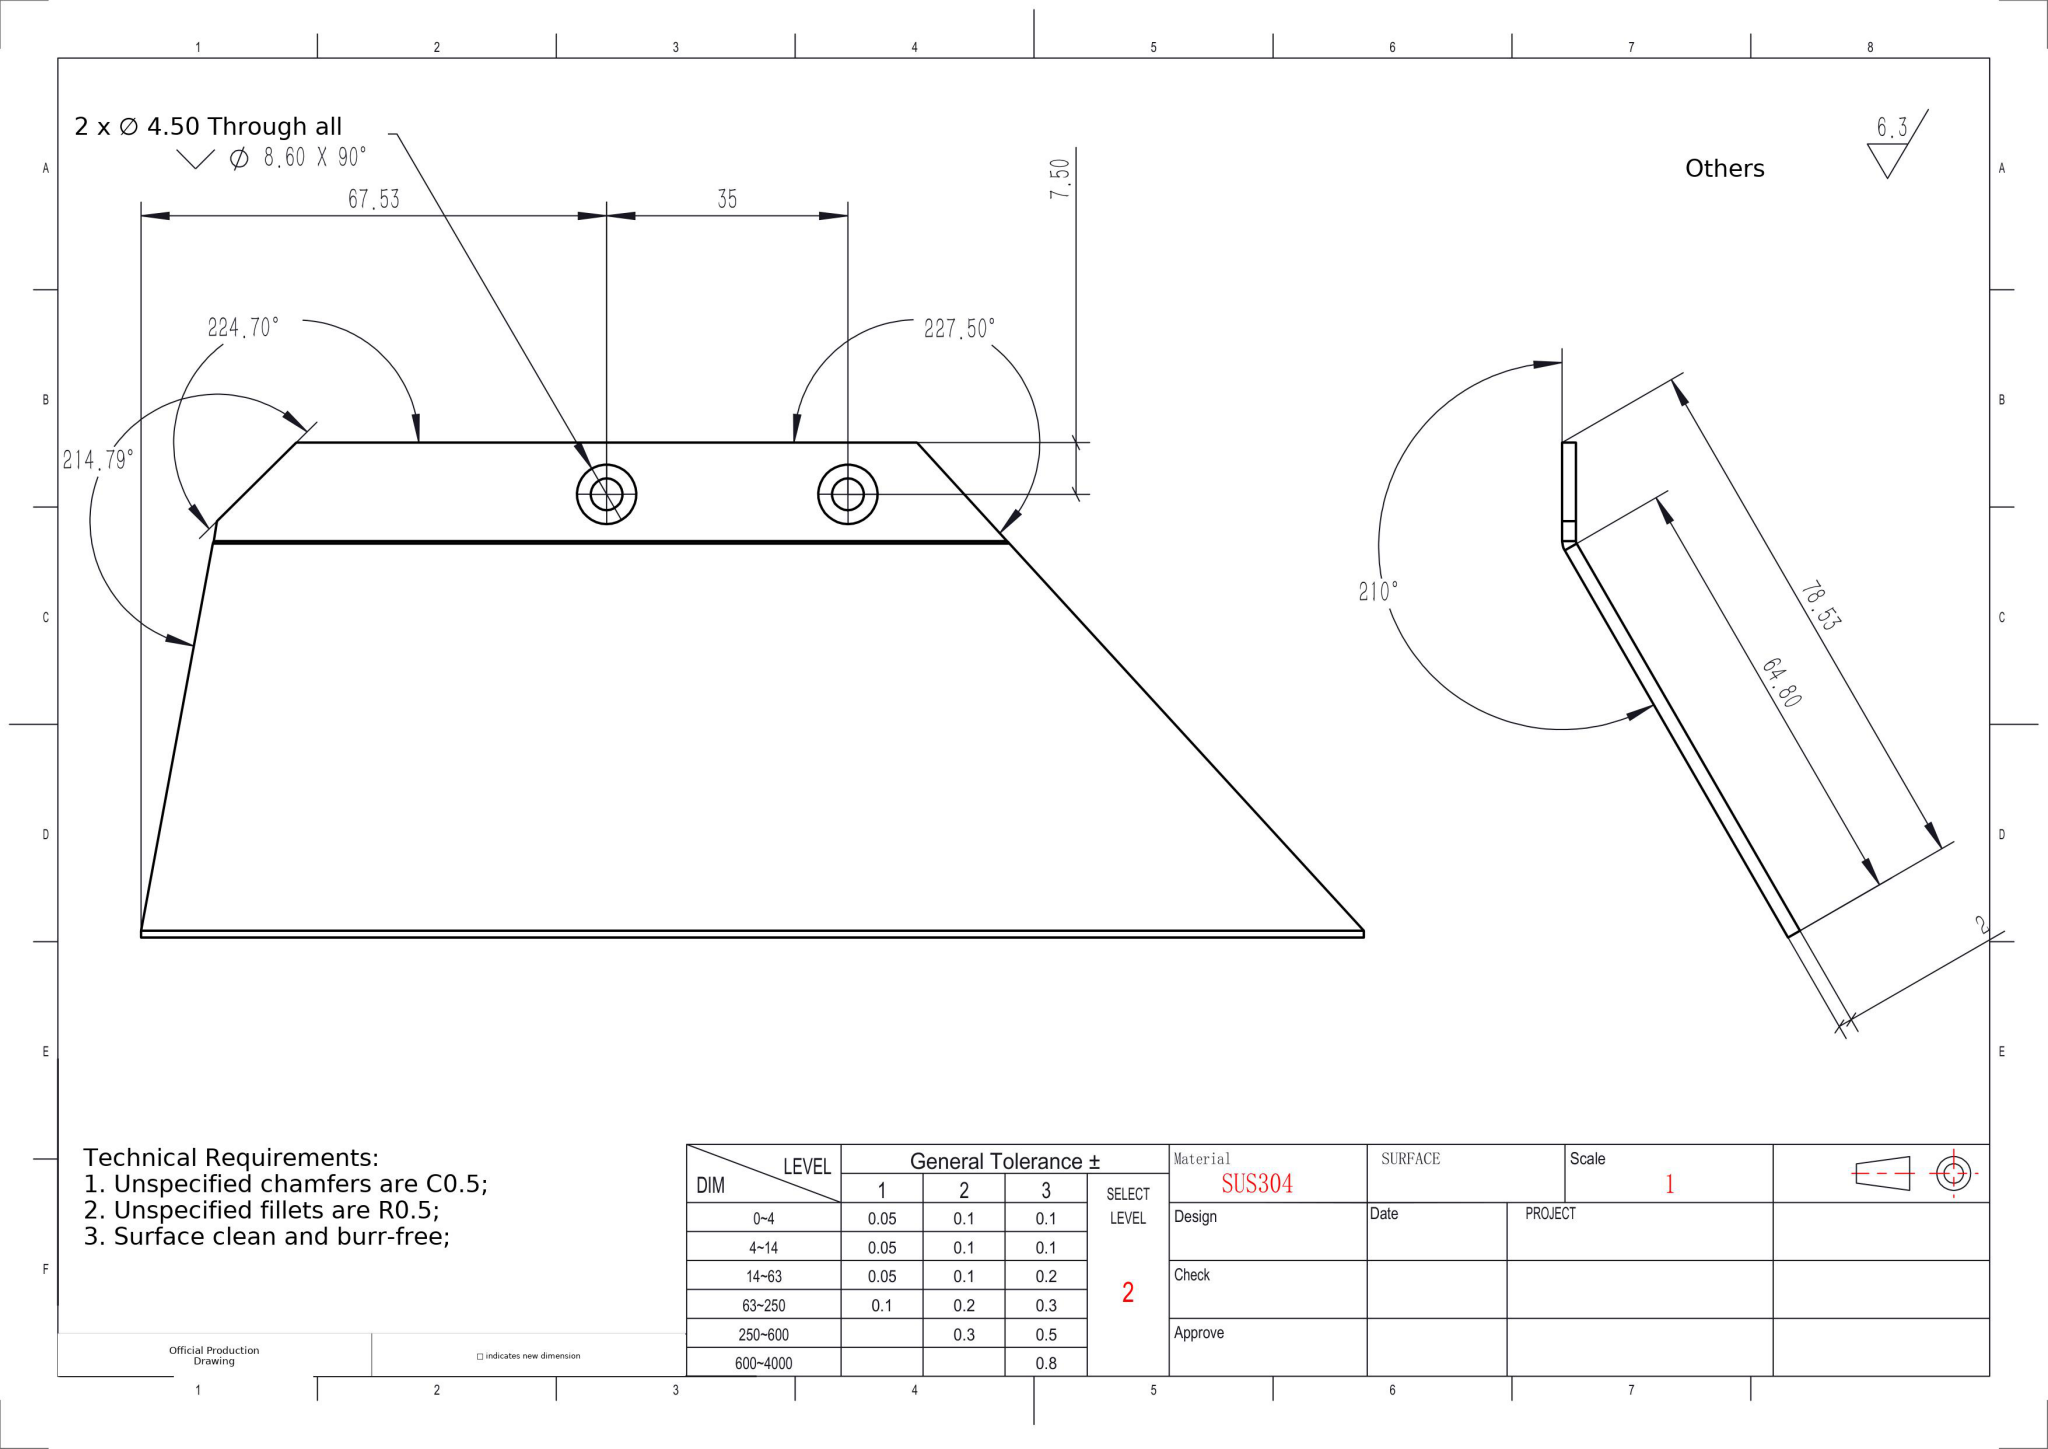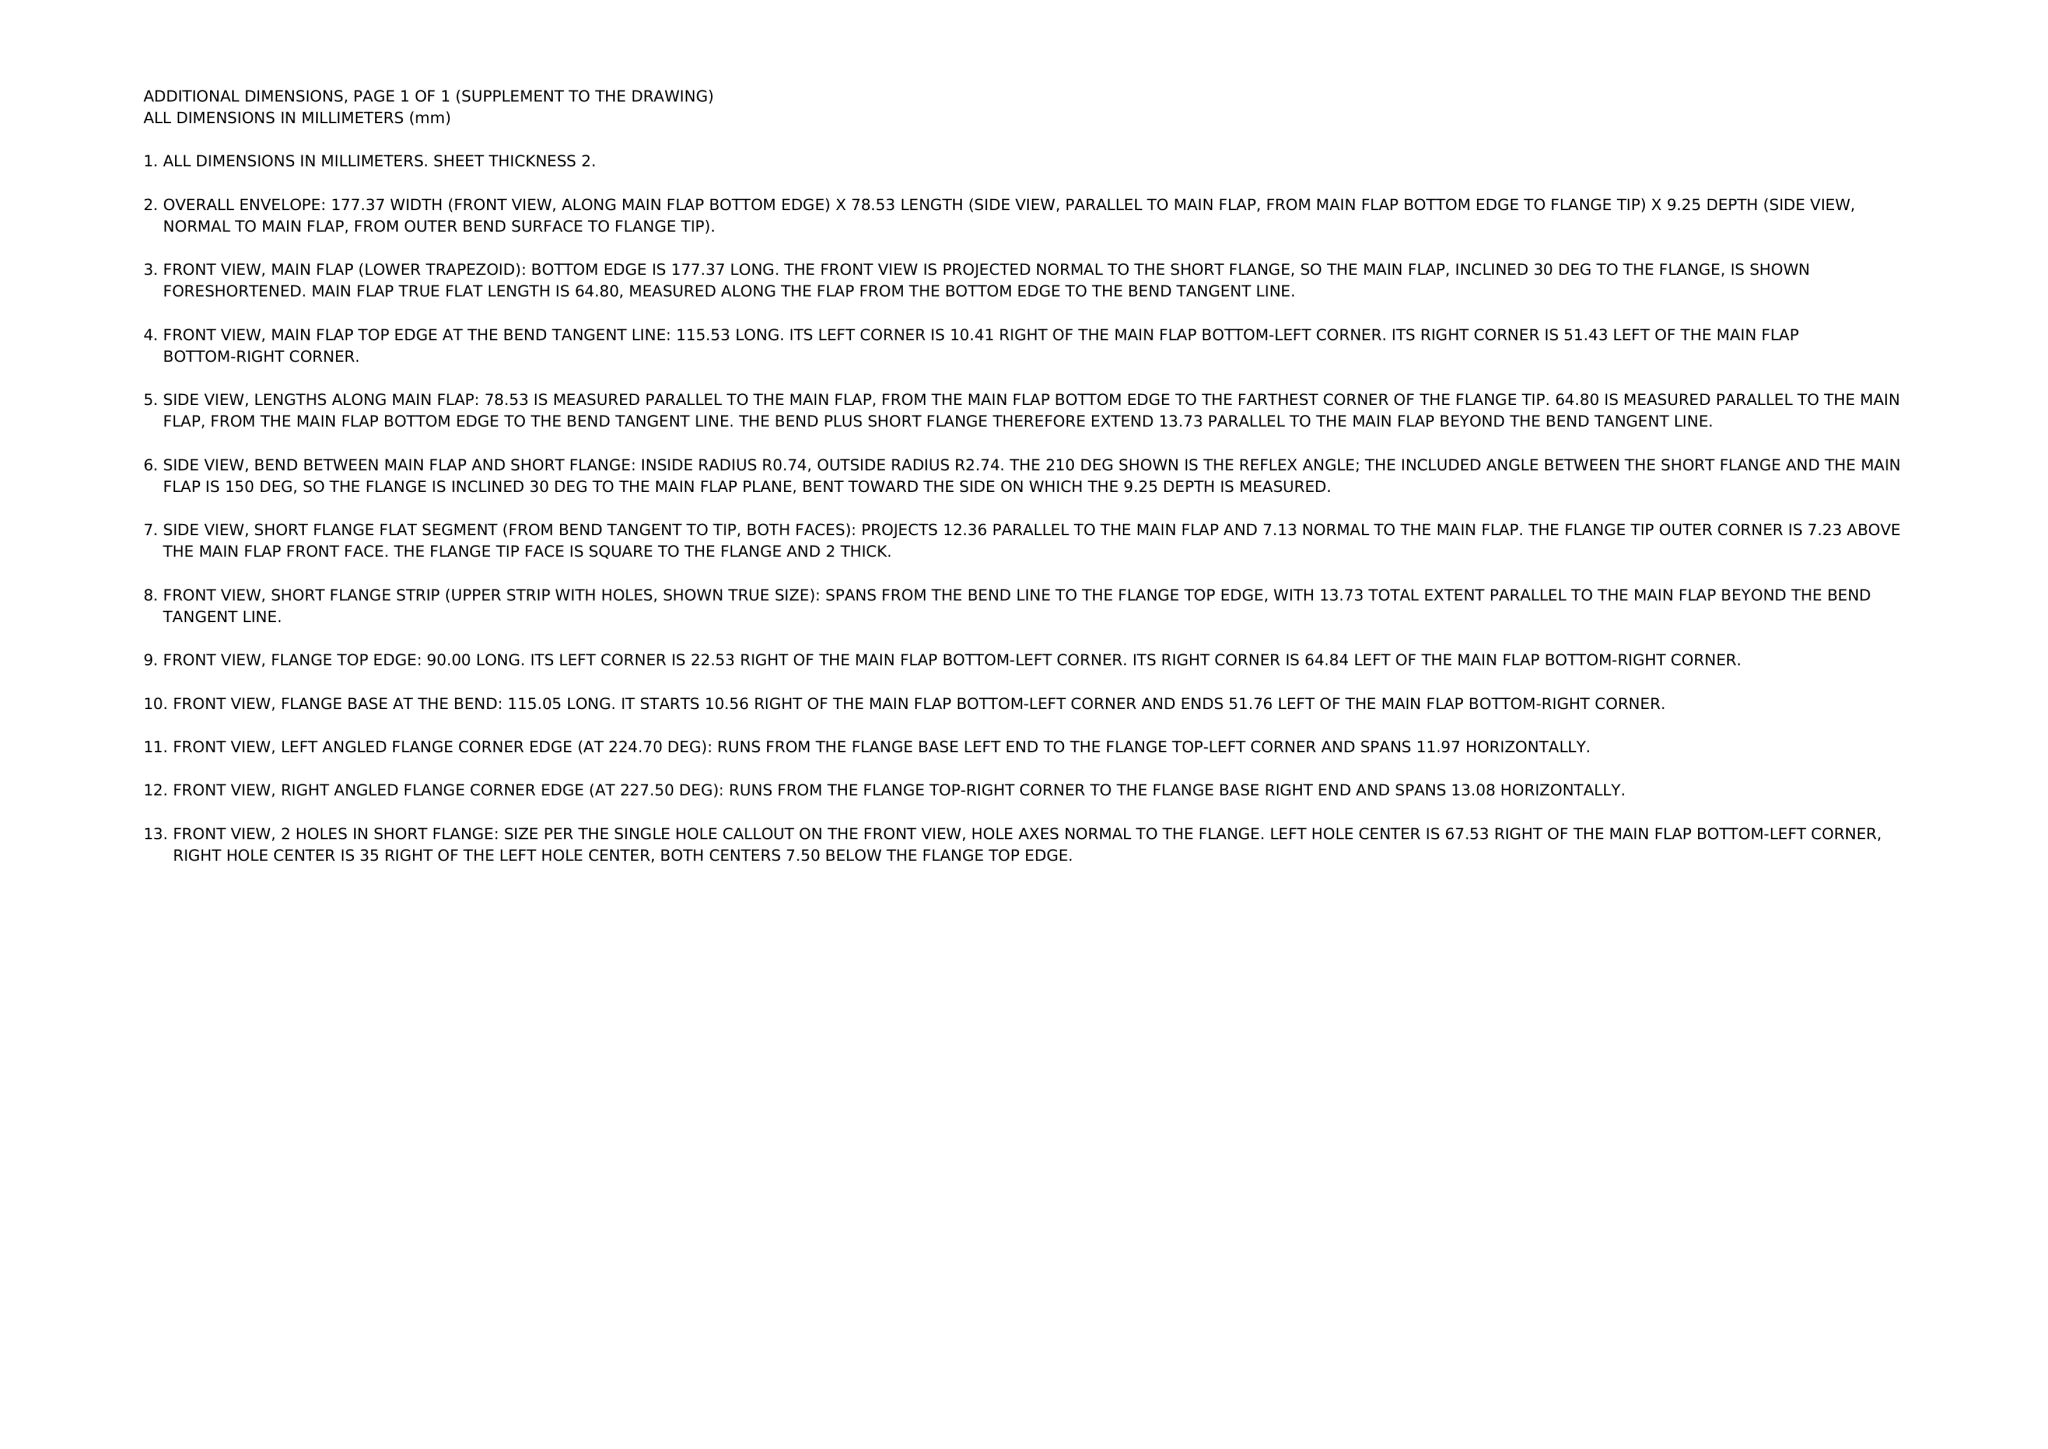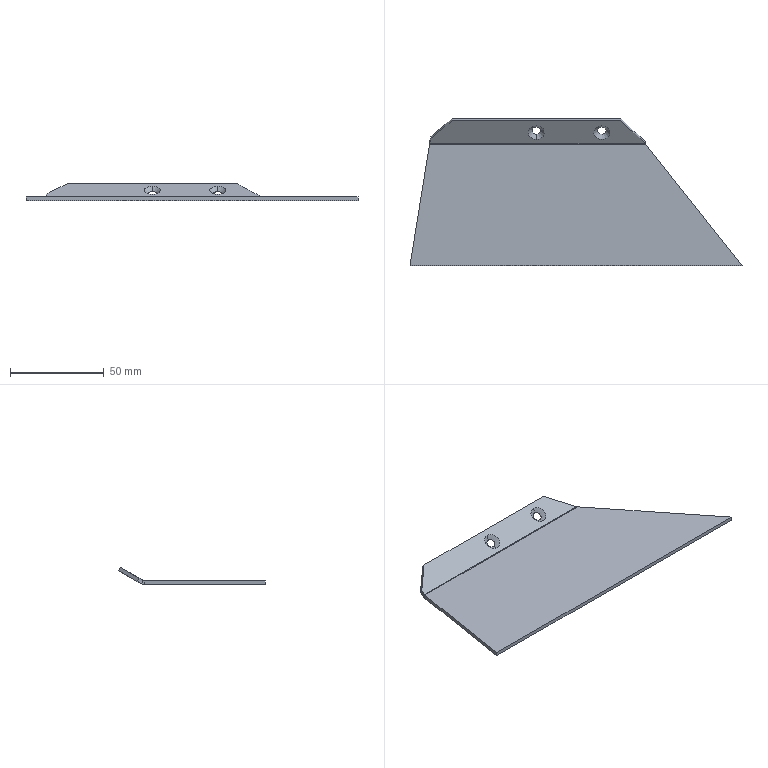Part | NX | mm | 1 solid | 19 faces | box 177.37 x 78.53 x 9.23 mm | volume 22003 mm3 | plane 11 | cone 4 | cylinder 2 | spline 2 | commonest cylinder face diameters 5.473 x1 1.473 x1
STEP:
#1=COLOUR_RGB('',0.698,0.698,0.698);
#2=FILL_AREA_STYLE_COLOUR('',#1);
#3=FILL_AREA_STYLE('',(#2));
#4=SURFACE_STYLE_FILL_AREA(#3);
#5=SURFACE_SIDE_STYLE('',(#4));
#6=SURFACE_STYLE_USAGE(.BOTH.,#5);
#7=PRESENTATION_STYLE_ASSIGNMENT((#6));
#8=CARTESIAN_POINT('',(25.164,41.523,2.9));
#9=VERTEX_POINT('',#8);
#10=CARTESIAN_POINT('',(25.164,37.539,0.6));
#11=VERTEX_POINT('',#10);
#12=CARTESIAN_POINT('',(25.164,39.531,1.75));
#13=DIRECTION('',(0.,-0.5,0.866));
#14=DIRECTION('',(0.,-0.866,-0.5));
#15=AXIS2_PLACEMENT_3D('',#12,#13,#14);
#16=CIRCLE('',#15,2.3);
#17=EDGE_CURVE('',#9,#11,#16,.T.);
#18=ORIENTED_EDGE('',*,*,#17,.F.);
#19=CARTESIAN_POINT('',(25.164,42.255,5.632));
#20=VERTEX_POINT('',#19);
#21=CARTESIAN_POINT('',(25.164,42.255,5.632));
#22=DIRECTION('',(0.,0.2588,0.9659));
#23=VECTOR('',#22,1000.);
#24=LINE('',#21,#23);
#25=EDGE_CURVE('',#9,#20,#24,.T.);
#26=ORIENTED_EDGE('',*,*,#25,.T.);
#27=CARTESIAN_POINT('',(25.164,34.807,1.332));
#28=VERTEX_POINT('',#27);
#29=CARTESIAN_POINT('',(25.164,38.531,3.482));
#30=DIRECTION('',(0.,-0.5,0.866));
#31=DIRECTION('',(0.,-0.866,-0.5));
#32=AXIS2_PLACEMENT_3D('',#29,#30,#31);
#33=CIRCLE('',#32,4.3);
#34=EDGE_CURVE('',#20,#28,#33,.T.);
#35=ORIENTED_EDGE('',*,*,#34,.T.);
#36=CARTESIAN_POINT('',(25.164,34.807,1.332));
#37=DIRECTION('',(0.,-0.9659,0.2588));
#38=VECTOR('',#37,1000.);
#39=LINE('',#36,#38);
#40=EDGE_CURVE('',#11,#28,#39,.T.);
#41=ORIENTED_EDGE('',*,*,#40,.F.);
#42=EDGE_LOOP('',(#18,#26,#35,#41));
#43=FACE_OUTER_BOUND('',#42,.T.);
#44=CARTESIAN_POINT('',(25.164,38.531,3.482));
#45=DIRECTION('',(0.,-0.5,0.866));
#46=DIRECTION('',(0.,-0.866,-0.5));
#47=AXIS2_PLACEMENT_3D('',#44,#45,#46);
#48=CONICAL_SURFACE('',#47,4.3,0.7854);
#49=ADVANCED_FACE('',(#43),#48,.F.);
#50=CARTESIAN_POINT('',(-9.836,41.523,2.9));
#51=VERTEX_POINT('',#50);
#52=CARTESIAN_POINT('',(-9.836,37.539,0.6));
#53=VERTEX_POINT('',#52);
#54=CARTESIAN_POINT('',(-9.836,39.531,1.75));
#55=DIRECTION('',(0.,-0.5,0.866));
#56=DIRECTION('',(0.,-0.866,-0.5));
#57=AXIS2_PLACEMENT_3D('',#54,#55,#56);
#58=CIRCLE('',#57,2.3);
#59=EDGE_CURVE('',#51,#53,#58,.T.);
#60=ORIENTED_EDGE('',*,*,#59,.F.);
#61=CARTESIAN_POINT('',(-9.836,42.255,5.632));
#62=VERTEX_POINT('',#61);
#63=CARTESIAN_POINT('',(-9.836,42.255,5.632));
#64=DIRECTION('',(0.,0.2588,0.9659));
#65=VECTOR('',#64,1000.);
#66=LINE('',#63,#65);
#67=EDGE_CURVE('',#51,#62,#66,.T.);
#68=ORIENTED_EDGE('',*,*,#67,.T.);
#69=CARTESIAN_POINT('',(-9.836,34.807,1.332));
#70=VERTEX_POINT('',#69);
#71=CARTESIAN_POINT('',(-9.836,38.531,3.482));
#72=DIRECTION('',(0.,-0.5,0.866));
#73=DIRECTION('',(0.,-0.866,-0.5));
#74=AXIS2_PLACEMENT_3D('',#71,#72,#73);
#75=CIRCLE('',#74,4.3);
#76=EDGE_CURVE('',#62,#70,#75,.T.);
#77=ORIENTED_EDGE('',*,*,#76,.T.);
#78=CARTESIAN_POINT('',(-9.836,34.807,1.332));
#79=DIRECTION('',(0.,-0.9659,0.2588));
#80=VECTOR('',#79,1000.);
#81=LINE('',#78,#80);
#82=EDGE_CURVE('',#53,#70,#81,.T.);
#83=ORIENTED_EDGE('',*,*,#82,.F.);
#84=EDGE_LOOP('',(#60,#68,#77,#83));
#85=FACE_OUTER_BOUND('',#84,.T.);
#86=CARTESIAN_POINT('',(-9.836,38.531,3.482));
#87=DIRECTION('',(0.,-0.5,0.866));
#88=DIRECTION('',(0.,-0.866,-0.5));
#89=AXIS2_PLACEMENT_3D('',#86,#87,#88);
#90=CONICAL_SURFACE('',#89,4.3,0.7854);
#91=ADVANCED_FACE('',(#85),#90,.F.);
#92=CARTESIAN_POINT('',(-77.367,-32.5,-2.));
#93=VERTEX_POINT('',#92);
#94=CARTESIAN_POINT('',(-66.958,32.303,-2.));
#95=VERTEX_POINT('',#94);
#96=CARTESIAN_POINT('',(-70.332,11.298,-2.));
#97=DIRECTION('',(0.1586,0.9873,0.));
#98=VECTOR('',#97,1000.);
#99=LINE('',#96,#98);
#100=EDGE_CURVE('',#93,#95,#99,.T.);
#101=ORIENTED_EDGE('',*,*,#100,.T.);
#102=CARTESIAN_POINT('',(48.575,32.303,-2.));
#103=VERTEX_POINT('',#102);
#104=CARTESIAN_POINT('',(-100.,32.303,-2.));
#105=DIRECTION('',(1.,0.,0.));
#106=VECTOR('',#105,1000.);
#107=LINE('',#104,#106);
#108=EDGE_CURVE('',#95,#103,#107,.T.);
#109=ORIENTED_EDGE('',*,*,#108,.T.);
#110=CARTESIAN_POINT('',(100.,-32.5,-2.));
#111=VERTEX_POINT('',#110);
#112=CARTESIAN_POINT('',(45.534,36.134,-2.));
#113=DIRECTION('',(-0.6216,0.7833,0.));
#114=VECTOR('',#113,1000.);
#115=LINE('',#112,#114);
#116=EDGE_CURVE('',#111,#103,#115,.T.);
#117=ORIENTED_EDGE('',*,*,#116,.F.);
#118=CARTESIAN_POINT('',(-100.,-32.5,-2.));
#119=DIRECTION('',(1.,0.,0.));
#120=VECTOR('',#119,1000.);
#121=LINE('',#118,#120);
#122=EDGE_CURVE('',#93,#111,#121,.T.);
#123=ORIENTED_EDGE('',*,*,#122,.F.);
#124=EDGE_LOOP('',(#101,#109,#117,#123));
#125=FACE_OUTER_BOUND('',#124,.T.);
#126=CARTESIAN_POINT('',(0.,0.,-2.));
#127=DIRECTION('',(0.,0.,1.));
#128=DIRECTION('',(1.,0.,0.));
#129=AXIS2_PLACEMENT_3D('',#126,#127,#128);
#130=PLANE('',#129);
#131=ADVANCED_FACE('',(#125),#130,.F.);
#132=CARTESIAN_POINT('',(-66.958,32.303,-0.));
#133=VERTEX_POINT('',#132);
#134=CARTESIAN_POINT('',(48.575,32.303,0.));
#135=VERTEX_POINT('',#134);
#136=CARTESIAN_POINT('',(-100.,32.303,-0.));
#137=DIRECTION('',(1.,0.,0.));
#138=VECTOR('',#137,1000.);
#139=LINE('',#136,#138);
#140=EDGE_CURVE('',#133,#135,#139,.T.);
#141=ORIENTED_EDGE('',*,*,#140,.F.);
#142=CARTESIAN_POINT('',(-77.367,-32.5,0.));
#143=VERTEX_POINT('',#142);
#144=CARTESIAN_POINT('',(-70.332,11.298,0.));
#145=DIRECTION('',(0.1586,0.9873,0.));
#146=VECTOR('',#145,1000.);
#147=LINE('',#144,#146);
#148=EDGE_CURVE('',#143,#133,#147,.T.);
#149=ORIENTED_EDGE('',*,*,#148,.F.);
#150=CARTESIAN_POINT('',(100.,-32.5,0.));
#151=VERTEX_POINT('',#150);
#152=CARTESIAN_POINT('',(-100.,-32.5,0.));
#153=DIRECTION('',(1.,0.,0.));
#154=VECTOR('',#153,1000.);
#155=LINE('',#152,#154);
#156=EDGE_CURVE('',#143,#151,#155,.T.);
#157=ORIENTED_EDGE('',*,*,#156,.T.);
#158=CARTESIAN_POINT('',(45.534,36.134,0.));
#159=DIRECTION('',(-0.6216,0.7833,0.));
#160=VECTOR('',#159,1000.);
#161=LINE('',#158,#160);
#162=EDGE_CURVE('',#151,#135,#161,.T.);
#163=ORIENTED_EDGE('',*,*,#162,.T.);
#164=EDGE_LOOP('',(#141,#149,#157,#163));
#165=FACE_OUTER_BOUND('',#164,.T.);
#166=CARTESIAN_POINT('',(0.,0.,0.));
#167=DIRECTION('',(0.,0.,1.));
#168=DIRECTION('',(1.,0.,0.));
#169=AXIS2_PLACEMENT_3D('',#166,#167,#168);
#170=PLANE('',#169);
#171=ADVANCED_FACE('',(#165),#170,.T.);
#172=ORIENTED_EDGE('',*,*,#108,.F.);
#173=CARTESIAN_POINT('',(-66.813,33.671,-1.633));
#174=VERTEX_POINT('',#173);
#175=CARTESIAN_POINT('',(-66.958,32.303,-2.));
#176=CARTESIAN_POINT('',(-66.934,32.542,-2.));
#177=CARTESIAN_POINT('',(-66.91,32.781,-1.969));
#178=CARTESIAN_POINT('',(-66.861,33.243,-1.844));
#179=CARTESIAN_POINT('',(-66.837,33.463,-1.753));
#180=CARTESIAN_POINT('',(-66.813,33.671,-1.633));
#181=B_SPLINE_CURVE_WITH_KNOTS('',3,(#175,#176,#177,#178,#179,#180),.UNSPECIFIED.,.F.,.F.,(4,2,4),(0.,0.0007209,0.001442),.UNSPECIFIED.);
#182=EDGE_CURVE('',#95,#174,#181,.T.);
#183=ORIENTED_EDGE('',*,*,#182,.T.);
#184=CARTESIAN_POINT('',(48.237,33.671,-1.633));
#185=VERTEX_POINT('',#184);
#186=CARTESIAN_POINT('',(0.,33.671,-1.633));
#187=DIRECTION('',(1.,0.,0.));
#188=VECTOR('',#187,1000.);
#189=LINE('',#186,#188);
#190=EDGE_CURVE('',#174,#185,#189,.T.);
#191=ORIENTED_EDGE('',*,*,#190,.T.);
#192=CARTESIAN_POINT('',(48.237,33.671,-1.633));
#193=CARTESIAN_POINT('',(48.294,33.463,-1.753));
#194=CARTESIAN_POINT('',(48.35,33.241,-1.845));
#195=CARTESIAN_POINT('',(48.463,32.778,-1.969));
#196=CARTESIAN_POINT('',(48.518,32.542,-2.));
#197=CARTESIAN_POINT('',(48.575,32.303,-2.));
#198=B_SPLINE_CURVE_WITH_KNOTS('',3,(#192,#193,#194,#195,#196,#197),.UNSPECIFIED.,.F.,.F.,(4,2,4),(0.,0.0007368,0.001474),.UNSPECIFIED.);
#199=EDGE_CURVE('',#185,#103,#198,.T.);
#200=ORIENTED_EDGE('',*,*,#199,.T.);
#201=EDGE_LOOP('',(#172,#183,#191,#200));
#202=FACE_OUTER_BOUND('',#201,.T.);
#203=CARTESIAN_POINT('',(-100.,32.303,0.7366));
#204=DIRECTION('',(-1.,0.,-0.));
#205=DIRECTION('',(0.,0.5,-0.866));
#206=AXIS2_PLACEMENT_3D('',#203,#204,#205);
#207=CYLINDRICAL_SURFACE('',#206,2.737);
#208=ADVANCED_FACE('',(#202),#207,.T.);
#209=CARTESIAN_POINT('',(-66.813,32.671,0.09869));
#210=VERTEX_POINT('',#209);
#211=CARTESIAN_POINT('',(-66.958,32.303,-0.));
#212=CARTESIAN_POINT('',(-66.91,32.432,-0.));
#213=CARTESIAN_POINT('',(-66.862,32.559,0.03421));
#214=CARTESIAN_POINT('',(-66.813,32.671,0.09869));
#215=B_SPLINE_CURVE_WITH_KNOTS('',3,(#211,#212,#213,#214),.UNSPECIFIED.,.F.,.F.,(4,4),(0.,0.0004102),.UNSPECIFIED.);
#216=EDGE_CURVE('',#133,#210,#215,.T.);
#217=ORIENTED_EDGE('',*,*,#216,.F.);
#218=ORIENTED_EDGE('',*,*,#140,.T.);
#219=CARTESIAN_POINT('',(48.237,32.671,0.09869));
#220=VERTEX_POINT('',#219);
#221=CARTESIAN_POINT('',(48.237,32.671,0.09869));
#222=CARTESIAN_POINT('',(48.35,32.559,0.03431));
#223=CARTESIAN_POINT('',(48.462,32.431,-0.));
#224=CARTESIAN_POINT('',(48.575,32.303,0.));
#225=B_SPLINE_CURVE_WITH_KNOTS('',3,(#221,#222,#223,#224),.UNSPECIFIED.,.F.,.F.,(4,4),(0.,0.0005119),.UNSPECIFIED.);
#226=EDGE_CURVE('',#220,#135,#225,.T.);
#227=ORIENTED_EDGE('',*,*,#226,.F.);
#228=CARTESIAN_POINT('',(100.,32.671,0.09869));
#229=DIRECTION('',(-1.,0.,0.));
#230=VECTOR('',#229,1000.);
#231=LINE('',#228,#230);
#232=EDGE_CURVE('',#220,#210,#231,.T.);
#233=ORIENTED_EDGE('',*,*,#232,.T.);
#234=EDGE_LOOP('',(#217,#218,#227,#233));
#235=FACE_OUTER_BOUND('',#234,.T.);
#236=CARTESIAN_POINT('',(-100.,32.303,0.7366));
#237=DIRECTION('',(-1.,0.,-0.));
#238=DIRECTION('',(0.,0.5,-0.866));
#239=AXIS2_PLACEMENT_3D('',#236,#237,#238);
#240=CYLINDRICAL_SURFACE('',#239,0.7366);
#241=ADVANCED_FACE('',(#235),#240,.F.);
#242=CARTESIAN_POINT('',(25.164,39.531,1.75));
#243=DIRECTION('',(0.,-0.5,0.866));
#244=DIRECTION('',(0.,-0.866,-0.5));
#245=AXIS2_PLACEMENT_3D('',#242,#243,#244);
#246=CIRCLE('',#245,2.3);
#247=EDGE_CURVE('',#11,#9,#246,.T.);
#248=ORIENTED_EDGE('',*,*,#247,.T.);
#249=ORIENTED_EDGE('',*,*,#17,.T.);
#250=EDGE_LOOP('',(#248,#249));
#251=FACE_BOUND('',#250,.T.);
#252=CARTESIAN_POINT('',(-9.836,39.531,1.75));
#253=DIRECTION('',(0.,-0.5,0.866));
#254=DIRECTION('',(0.,-0.866,-0.5));
#255=AXIS2_PLACEMENT_3D('',#252,#253,#254);
#256=CIRCLE('',#255,2.3);
#257=EDGE_CURVE('',#53,#51,#256,.T.);
#258=ORIENTED_EDGE('',*,*,#257,.T.);
#259=ORIENTED_EDGE('',*,*,#59,.T.);
#260=EDGE_LOOP('',(#258,#259));
#261=FACE_BOUND('',#260,.T.);
#262=CARTESIAN_POINT('',(-66.356,36.16,-0.1963));
#263=VERTEX_POINT('',#262);
#264=CARTESIAN_POINT('',(-66.356,36.16,-0.1963));
#265=DIRECTION('',(-0.157,-0.8553,-0.4938));
#266=VECTOR('',#265,1000.);
#267=LINE('',#264,#266);
#268=EDGE_CURVE('',#263,#174,#267,.T.);
#269=ORIENTED_EDGE('',*,*,#268,.F.);
#270=CARTESIAN_POINT('',(-54.844,46.026,5.5));
#271=VERTEX_POINT('',#270);
#272=CARTESIAN_POINT('',(-48.439,51.515,8.669));
#273=DIRECTION('',(0.7108,0.6092,0.3517));
#274=VECTOR('',#273,1000.);
#275=LINE('',#272,#274);
#276=EDGE_CURVE('',#263,#271,#275,.T.);
#277=ORIENTED_EDGE('',*,*,#276,.T.);
#278=CARTESIAN_POINT('',(35.164,46.026,5.5));
#279=VERTEX_POINT('',#278);
#280=CARTESIAN_POINT('',(100.,46.026,5.5));
#281=DIRECTION('',(1.,0.,0.));
#282=VECTOR('',#281,1000.);
#283=LINE('',#280,#282);
#284=EDGE_CURVE('',#271,#279,#283,.T.);
#285=ORIENTED_EDGE('',*,*,#284,.T.);
#286=CARTESIAN_POINT('',(40.338,41.136,2.677));
#287=DIRECTION('',(0.6756,-0.6385,-0.3686));
#288=VECTOR('',#287,1000.);
#289=LINE('',#286,#288);
#290=EDGE_CURVE('',#279,#185,#289,.T.);
#291=ORIENTED_EDGE('',*,*,#290,.T.);
#292=ORIENTED_EDGE('',*,*,#190,.F.);
#293=EDGE_LOOP('',(#269,#277,#285,#291,#292));
#294=FACE_OUTER_BOUND('',#293,.T.);
#295=CARTESIAN_POINT('',(0.,9.125,-15.805));
#296=DIRECTION('',(0.,-0.5,0.866));
#297=DIRECTION('',(0.,-0.866,-0.5));
#298=AXIS2_PLACEMENT_3D('',#295,#296,#297);
#299=PLANE('',#298);
#300=ADVANCED_FACE('',(#251,#261,#294),#299,.F.);
#301=CARTESIAN_POINT('',(25.164,38.531,3.482));
#302=DIRECTION('',(0.,-0.5,0.866));
#303=DIRECTION('',(0.,-0.866,-0.5));
#304=AXIS2_PLACEMENT_3D('',#301,#302,#303);
#305=CIRCLE('',#304,4.3);
#306=EDGE_CURVE('',#28,#20,#305,.T.);
#307=ORIENTED_EDGE('',*,*,#306,.F.);
#308=ORIENTED_EDGE('',*,*,#34,.F.);
#309=EDGE_LOOP('',(#307,#308));
#310=FACE_BOUND('',#309,.T.);
#311=CARTESIAN_POINT('',(-9.836,38.531,3.482));
#312=DIRECTION('',(0.,-0.5,0.866));
#313=DIRECTION('',(0.,-0.866,-0.5));
#314=AXIS2_PLACEMENT_3D('',#311,#312,#313);
#315=CIRCLE('',#314,4.3);
#316=EDGE_CURVE('',#70,#62,#315,.T.);
#317=ORIENTED_EDGE('',*,*,#316,.F.);
#318=ORIENTED_EDGE('',*,*,#76,.F.);
#319=EDGE_LOOP('',(#317,#318));
#320=FACE_BOUND('',#319,.T.);
#321=CARTESIAN_POINT('',(-66.356,35.16,1.536));
#322=VERTEX_POINT('',#321);
#323=CARTESIAN_POINT('',(-54.844,45.026,7.232));
#324=VERTEX_POINT('',#323);
#325=CARTESIAN_POINT('',(-48.439,50.515,10.401));
#326=DIRECTION('',(0.7108,0.6092,0.3517));
#327=VECTOR('',#326,1000.);
#328=LINE('',#325,#327);
#329=EDGE_CURVE('',#322,#324,#328,.T.);
#330=ORIENTED_EDGE('',*,*,#329,.F.);
#331=CARTESIAN_POINT('',(-66.356,35.16,1.536));
#332=DIRECTION('',(-0.157,-0.8553,-0.4938));
#333=VECTOR('',#332,1000.);
#334=LINE('',#331,#333);
#335=EDGE_CURVE('',#322,#210,#334,.T.);
#336=ORIENTED_EDGE('',*,*,#335,.T.);
#337=ORIENTED_EDGE('',*,*,#232,.F.);
#338=CARTESIAN_POINT('',(35.164,45.026,7.232));
#339=VERTEX_POINT('',#338);
#340=CARTESIAN_POINT('',(40.338,40.136,4.409));
#341=DIRECTION('',(0.6756,-0.6385,-0.3686));
#342=VECTOR('',#341,1000.);
#343=LINE('',#340,#342);
#344=EDGE_CURVE('',#339,#220,#343,.T.);
#345=ORIENTED_EDGE('',*,*,#344,.F.);
#346=CARTESIAN_POINT('',(100.,45.026,7.232));
#347=DIRECTION('',(1.,0.,0.));
#348=VECTOR('',#347,1000.);
#349=LINE('',#346,#348);
#350=EDGE_CURVE('',#324,#339,#349,.T.);
#351=ORIENTED_EDGE('',*,*,#350,.F.);
#352=EDGE_LOOP('',(#330,#336,#337,#345,#351));
#353=FACE_OUTER_BOUND('',#352,.T.);
#354=CARTESIAN_POINT('',(0.,8.125,-14.073));
#355=DIRECTION('',(0.,-0.5,0.866));
#356=DIRECTION('',(0.,-0.866,-0.5));
#357=AXIS2_PLACEMENT_3D('',#354,#355,#356);
#358=PLANE('',#357);
#359=ADVANCED_FACE('',(#310,#320,#353),#358,.T.);
#360=CARTESIAN_POINT('',(-54.844,45.026,7.232));
#361=DIRECTION('',(0.,0.5,-0.866));
#362=VECTOR('',#361,1000.);
#363=LINE('',#360,#362);
#364=EDGE_CURVE('',#324,#271,#363,.T.);
#365=ORIENTED_EDGE('',*,*,#364,.F.);
#366=ORIENTED_EDGE('',*,*,#350,.T.);
#367=CARTESIAN_POINT('',(35.164,46.026,5.5));
#368=DIRECTION('',(0.,0.5,-0.866));
#369=VECTOR('',#368,1000.);
#370=LINE('',#367,#369);
#371=EDGE_CURVE('',#339,#279,#370,.T.);
#372=ORIENTED_EDGE('',*,*,#371,.T.);
#373=ORIENTED_EDGE('',*,*,#284,.F.);
#374=EDGE_LOOP('',(#365,#366,#372,#373));
#375=FACE_OUTER_BOUND('',#374,.T.);
#376=CARTESIAN_POINT('',(100.,46.026,5.5));
#377=DIRECTION('',(0.,-0.866,-0.5));
#378=DIRECTION('',(0.,0.5,-0.866));
#379=AXIS2_PLACEMENT_3D('',#376,#377,#378);
#380=PLANE('',#379);
#381=ADVANCED_FACE('',(#375),#380,.F.);
#382=ORIENTED_EDGE('',*,*,#156,.F.);
#383=CARTESIAN_POINT('',(-77.367,-32.5,0.));
#384=DIRECTION('',(0.,0.,-1.));
#385=VECTOR('',#384,1000.);
#386=LINE('',#383,#385);
#387=EDGE_CURVE('',#143,#93,#386,.T.);
#388=ORIENTED_EDGE('',*,*,#387,.T.);
#389=ORIENTED_EDGE('',*,*,#122,.T.);
#390=CARTESIAN_POINT('',(100.,-32.5,-2.));
#391=DIRECTION('',(0.,0.,1.));
#392=VECTOR('',#391,1000.);
#393=LINE('',#390,#392);
#394=EDGE_CURVE('',#111,#151,#393,.T.);
#395=ORIENTED_EDGE('',*,*,#394,.T.);
#396=EDGE_LOOP('',(#382,#388,#389,#395));
#397=FACE_OUTER_BOUND('',#396,.T.);
#398=CARTESIAN_POINT('',(-100.,-32.5,-2.));
#399=DIRECTION('',(0.,-1.,0.));
#400=DIRECTION('',(0.,0.,-1.));
#401=AXIS2_PLACEMENT_3D('',#398,#399,#400);
#402=PLANE('',#401);
#403=ADVANCED_FACE('',(#397),#402,.T.);
#404=ORIENTED_EDGE('',*,*,#371,.F.);
#405=ORIENTED_EDGE('',*,*,#344,.T.);
#406=CARTESIAN_POINT('',(48.237,33.671,-1.633));
#407=DIRECTION('',(-0.,-0.5,0.866));
#408=VECTOR('',#407,1000.);
#409=LINE('',#406,#408);
#410=EDGE_CURVE('',#185,#220,#409,.T.);
#411=ORIENTED_EDGE('',*,*,#410,.F.);
#412=ORIENTED_EDGE('',*,*,#290,.F.);
#413=EDGE_LOOP('',(#404,#405,#411,#412));
#414=FACE_OUTER_BOUND('',#413,.T.);
#415=CARTESIAN_POINT('',(40.338,41.136,2.677));
#416=DIRECTION('',(-0.7373,-0.5851,-0.3378));
#417=DIRECTION('',(0.6756,-0.6385,-0.3686));
#418=AXIS2_PLACEMENT_3D('',#415,#416,#417);
#419=PLANE('',#418);
#420=ADVANCED_FACE('',(#414),#419,.F.);
#421=ORIENTED_EDGE('',*,*,#410,.T.);
#422=ORIENTED_EDGE('',*,*,#226,.T.);
#423=CARTESIAN_POINT('',(48.575,32.303,0.));
#424=DIRECTION('',(0.,0.,1.));
#425=VECTOR('',#424,1000.);
#426=LINE('',#423,#425);
#427=EDGE_CURVE('',#103,#135,#426,.T.);
#428=ORIENTED_EDGE('',*,*,#427,.F.);
#429=ORIENTED_EDGE('',*,*,#199,.F.);
#430=EDGE_LOOP('',(#421,#422,#428,#429));
#431=FACE_OUTER_BOUND('',#430,.T.);
#432=CARTESIAN_POINT('',(48.237,33.681,-1.651));
#433=CARTESIAN_POINT('',(48.35,33.264,-1.892));
#434=CARTESIAN_POINT('',(48.462,32.784,-2.02));
#435=CARTESIAN_POINT('',(48.575,32.303,-2.02));
#436=CARTESIAN_POINT('',(48.237,33.671,-1.633));
#437=CARTESIAN_POINT('',(48.35,33.257,-1.873));
#438=CARTESIAN_POINT('',(48.462,32.781,-2.));
#439=CARTESIAN_POINT('',(48.575,32.303,-2.));
#440=CARTESIAN_POINT('',(48.237,32.671,0.09869));
#441=CARTESIAN_POINT('',(48.35,32.559,0.03434));
#442=CARTESIAN_POINT('',(48.462,32.431,-0.));
#443=CARTESIAN_POINT('',(48.575,32.303,-0.));
#444=B_SPLINE_SURFACE_WITH_KNOTS('',1,3,((#432,#433,#434,#435),(#436,#437,#438,#439),(#440,#441,#442,#443)),.UNSPECIFIED.,.F.,.F.,.F.,(2,1,2),(4,4),(-0.01,0.,1.),(0.,1.),.UNSPECIFIED.);
#445=ADVANCED_FACE('',(#431),#444,.T.);
#446=ORIENTED_EDGE('',*,*,#394,.F.);
#447=ORIENTED_EDGE('',*,*,#116,.T.);
#448=ORIENTED_EDGE('',*,*,#427,.T.);
#449=ORIENTED_EDGE('',*,*,#162,.F.);
#450=EDGE_LOOP('',(#446,#447,#448,#449));
#451=FACE_OUTER_BOUND('',#450,.T.);
#452=CARTESIAN_POINT('',(45.534,36.134,0.));
#453=DIRECTION('',(-0.7833,-0.6216,0.));
#454=DIRECTION('',(-0.6216,0.7833,0.));
#455=AXIS2_PLACEMENT_3D('',#452,#453,#454);
#456=PLANE('',#455);
#457=ADVANCED_FACE('',(#451),#456,.F.);
#458=CARTESIAN_POINT('',(-66.958,32.303,0.));
#459=DIRECTION('',(0.,0.,1.));
#460=VECTOR('',#459,1000.);
#461=LINE('',#458,#460);
#462=EDGE_CURVE('',#95,#133,#461,.T.);
#463=ORIENTED_EDGE('',*,*,#462,.T.);
#464=ORIENTED_EDGE('',*,*,#216,.T.);
#465=CARTESIAN_POINT('',(-66.813,32.671,0.09869));
#466=DIRECTION('',(0.,0.5,-0.866));
#467=VECTOR('',#466,1000.);
#468=LINE('',#465,#467);
#469=EDGE_CURVE('',#210,#174,#468,.T.);
#470=ORIENTED_EDGE('',*,*,#469,.T.);
#471=ORIENTED_EDGE('',*,*,#182,.F.);
#472=EDGE_LOOP('',(#463,#464,#470,#471));
#473=FACE_OUTER_BOUND('',#472,.T.);
#474=CARTESIAN_POINT('',(-66.958,32.303,-2.02));
#475=CARTESIAN_POINT('',(-66.91,32.785,-2.02));
#476=CARTESIAN_POINT('',(-66.862,33.264,-1.892));
#477=CARTESIAN_POINT('',(-66.813,33.681,-1.651));
#478=CARTESIAN_POINT('',(-66.958,32.303,-2.));
#479=CARTESIAN_POINT('',(-66.91,32.781,-2.));
#480=CARTESIAN_POINT('',(-66.862,33.257,-1.873));
#481=CARTESIAN_POINT('',(-66.813,33.671,-1.633));
#482=CARTESIAN_POINT('',(-66.958,32.303,-0.));
#483=CARTESIAN_POINT('',(-66.91,32.431,-0.));
#484=CARTESIAN_POINT('',(-66.862,32.559,0.03431));
#485=CARTESIAN_POINT('',(-66.813,32.671,0.09869));
#486=B_SPLINE_SURFACE_WITH_KNOTS('',1,3,((#474,#475,#476,#477),(#478,#479,#480,#481),(#482,#483,#484,#485)),.UNSPECIFIED.,.F.,.F.,.F.,(2,1,2),(4,4),(-0.01,0.,1.),(0.,1.),.UNSPECIFIED.);
#487=ADVANCED_FACE('',(#473),#486,.T.);
#488=ORIENTED_EDGE('',*,*,#148,.T.);
#489=ORIENTED_EDGE('',*,*,#462,.F.);
#490=ORIENTED_EDGE('',*,*,#100,.F.);
#491=ORIENTED_EDGE('',*,*,#387,.F.);
#492=EDGE_LOOP('',(#488,#489,#490,#491));
#493=FACE_OUTER_BOUND('',#492,.T.);
#494=CARTESIAN_POINT('',(-70.332,11.298,0.));
#495=DIRECTION('',(0.9873,-0.1586,0.));
#496=DIRECTION('',(0.1586,0.9873,0.));
#497=AXIS2_PLACEMENT_3D('',#494,#495,#496);
#498=PLANE('',#497);
#499=ADVANCED_FACE('',(#493),#498,.F.);
#500=ORIENTED_EDGE('',*,*,#469,.F.);
#501=ORIENTED_EDGE('',*,*,#335,.F.);
#502=CARTESIAN_POINT('',(-66.356,35.16,1.536));
#503=DIRECTION('',(0.,0.5,-0.866));
#504=VECTOR('',#503,1000.);
#505=LINE('',#502,#504);
#506=EDGE_CURVE('',#322,#263,#505,.T.);
#507=ORIENTED_EDGE('',*,*,#506,.T.);
#508=ORIENTED_EDGE('',*,*,#268,.T.);
#509=EDGE_LOOP('',(#500,#501,#507,#508));
#510=FACE_OUTER_BOUND('',#509,.T.);
#511=CARTESIAN_POINT('',(-66.356,35.16,1.536));
#512=DIRECTION('',(0.9876,-0.136,-0.0785));
#513=DIRECTION('',(-0.157,-0.8553,-0.4938));
#514=AXIS2_PLACEMENT_3D('',#511,#512,#513);
#515=PLANE('',#514);
#516=ADVANCED_FACE('',(#510),#515,.F.);
#517=ORIENTED_EDGE('',*,*,#506,.F.);
#518=ORIENTED_EDGE('',*,*,#329,.T.);
#519=ORIENTED_EDGE('',*,*,#364,.T.);
#520=ORIENTED_EDGE('',*,*,#276,.F.);
#521=EDGE_LOOP('',(#517,#518,#519,#520));
#522=FACE_OUTER_BOUND('',#521,.T.);
#523=CARTESIAN_POINT('',(-48.439,50.515,10.401));
#524=DIRECTION('',(0.7034,-0.6156,-0.3554));
#525=DIRECTION('',(0.7108,0.6092,0.3517));
#526=AXIS2_PLACEMENT_3D('',#523,#524,#525);
#527=PLANE('',#526);
#528=ADVANCED_FACE('',(#522),#527,.F.);
#529=ORIENTED_EDGE('',*,*,#67,.F.);
#530=ORIENTED_EDGE('',*,*,#257,.F.);
#531=ORIENTED_EDGE('',*,*,#82,.T.);
#532=ORIENTED_EDGE('',*,*,#316,.T.);
#533=EDGE_LOOP('',(#529,#530,#531,#532));
#534=FACE_OUTER_BOUND('',#533,.T.);
#535=CARTESIAN_POINT('',(-9.836,38.531,3.482));
#536=DIRECTION('',(0.,-0.5,0.866));
#537=DIRECTION('',(0.,-0.866,-0.5));
#538=AXIS2_PLACEMENT_3D('',#535,#536,#537);
#539=CONICAL_SURFACE('',#538,4.3,0.7854);
#540=ADVANCED_FACE('',(#534),#539,.F.);
#541=ORIENTED_EDGE('',*,*,#25,.F.);
#542=ORIENTED_EDGE('',*,*,#247,.F.);
#543=ORIENTED_EDGE('',*,*,#40,.T.);
#544=ORIENTED_EDGE('',*,*,#306,.T.);
#545=EDGE_LOOP('',(#541,#542,#543,#544));
#546=FACE_OUTER_BOUND('',#545,.T.);
#547=CARTESIAN_POINT('',(25.164,38.531,3.482));
#548=DIRECTION('',(0.,-0.5,0.866));
#549=DIRECTION('',(0.,-0.866,-0.5));
#550=AXIS2_PLACEMENT_3D('',#547,#548,#549);
#551=CONICAL_SURFACE('',#550,4.3,0.7854);
#552=ADVANCED_FACE('',(#546),#551,.F.);
#553=CLOSED_SHELL('',(#49,#91,#131,#171,#208,#241,#300,#359,#381,#403,#420,#445,#457,#487,#499,#516,#528,#540,#552));
#554=MANIFOLD_SOLID_BREP('',#553);
#555=CARTESIAN_POINT('',(0.,0.,0.));
#556=DIRECTION('',(0.,0.,1.));
#557=DIRECTION('',(1.,0.,0.));
#558=AXIS2_PLACEMENT_3D('',#555,#556,#557);
#559=(LENGTH_UNIT()NAMED_UNIT(*)SI_UNIT(.MILLI.,.METRE.));
#560=UNCERTAINTY_MEASURE_WITH_UNIT(LENGTH_MEASURE(0.00001),#559,'','');
#561=(NAMED_UNIT(*)PLANE_ANGLE_UNIT()SI_UNIT($,.RADIAN.));
#562=(NAMED_UNIT(*)SI_UNIT($,.STERADIAN.)SOLID_ANGLE_UNIT());
#563=(GEOMETRIC_REPRESENTATION_CONTEXT(3)GLOBAL_UNCERTAINTY_ASSIGNED_CONTEXT((#560))GLOBAL_UNIT_ASSIGNED_CONTEXT((#559,#561,#562))REPRESENTATION_CONTEXT('',''));
#564=ADVANCED_BREP_SHAPE_REPRESENTATION('',(#554,#558),#563);
#565=STYLED_ITEM('',(#7),#564);
#566=(LENGTH_UNIT()NAMED_UNIT(*)SI_UNIT(.MILLI.,.METRE.));
#567=UNCERTAINTY_MEASURE_WITH_UNIT(LENGTH_MEASURE(0.00001),#566,'','');
#568=(NAMED_UNIT(*)PLANE_ANGLE_UNIT()SI_UNIT($,.RADIAN.));
#569=(NAMED_UNIT(*)SI_UNIT($,.STERADIAN.)SOLID_ANGLE_UNIT());
#570=(GEOMETRIC_REPRESENTATION_CONTEXT(3)GLOBAL_UNCERTAINTY_ASSIGNED_CONTEXT((#567))GLOBAL_UNIT_ASSIGNED_CONTEXT((#566,#568,#569))REPRESENTATION_CONTEXT('',''));
#571=MECHANICAL_DESIGN_GEOMETRIC_PRESENTATION_REPRESENTATION('',(#565),#570);
#572=COLOUR_RGB('',0.698,0.698,0.698);
#573=FILL_AREA_STYLE_COLOUR('',#572);
#574=FILL_AREA_STYLE('',(#573));
#575=SURFACE_STYLE_FILL_AREA(#574);
#576=SURFACE_SIDE_STYLE('',(#575));
#577=SURFACE_STYLE_USAGE(.BOTH.,#576);
#578=PRESENTATION_STYLE_ASSIGNMENT((#577));
#579=STYLED_ITEM('',(#578),#554);
#580=PRESENTATION_LAYER_ASSIGNMENT('','',(#579));
#581=(LENGTH_UNIT()NAMED_UNIT(*)SI_UNIT(.MILLI.,.METRE.));
#582=UNCERTAINTY_MEASURE_WITH_UNIT(LENGTH_MEASURE(0.00001),#581,'','');
#583=(NAMED_UNIT(*)PLANE_ANGLE_UNIT()SI_UNIT($,.RADIAN.));
#584=(NAMED_UNIT(*)SI_UNIT($,.STERADIAN.)SOLID_ANGLE_UNIT());
#585=(GEOMETRIC_REPRESENTATION_CONTEXT(3)GLOBAL_UNCERTAINTY_ASSIGNED_CONTEXT((#582))GLOBAL_UNIT_ASSIGNED_CONTEXT((#581,#583,#584))REPRESENTATION_CONTEXT('',''));
#586=MECHANICAL_DESIGN_GEOMETRIC_PRESENTATION_REPRESENTATION('',(#579),#585);
#587=PRESENTATION_LAYER_ASSIGNMENT('','',(#565));